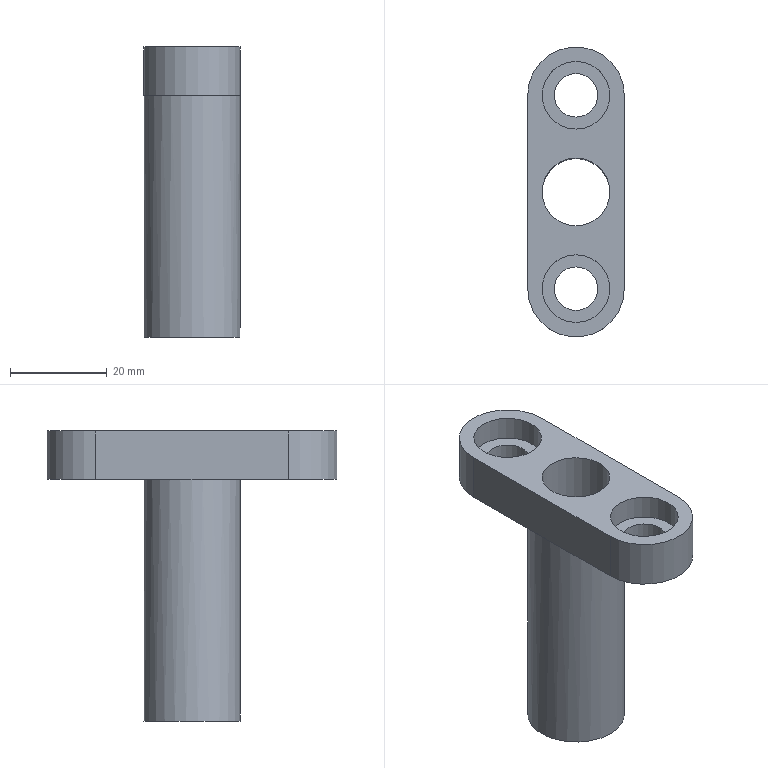Component | NX | GUIDE_BUSH | 1 solid | 16 faces | box 20 x 60 x 60 mm | volume 15438 mm3 | cylinder 8 | plane 8 | commonest cylinder face diameters 20 x3 14 x3 9 x2
STEP:
#1=CARTESIAN_POINT('',(0.,0.,0.));
#2=DIRECTION('',(0.,0.,1.));
#3=DIRECTION('',(1.,0.,0.));
#4=AXIS2_PLACEMENT_3D('',#1,#2,#3);
#5=CARTESIAN_POINT('',(40.594,327.962,290.466));
#6=VERTEX_POINT('',#5);
#7=CARTESIAN_POINT('',(40.594,332.462,290.466));
#8=DIRECTION('',(0.,0.,1.));
#9=DIRECTION('',(0.,-1.,0.));
#10=AXIS2_PLACEMENT_3D('',#7,#8,#9);
#11=CIRCLE('',#10,4.5);
#12=CARTESIAN_POINT('',(40.594,332.462,300.466));
#13=DIRECTION('',(0.,0.,-1.));
#14=DIRECTION('',(0.,1.,0.));
#15=AXIS2_PLACEMENT_3D('',#12,#13,#14);
#16=CYLINDRICAL_SURFACE('',#15,4.5);
#17=CARTESIAN_POINT('',(9.425,10.));
#18=DIRECTION('',(-1.,0.));
#19=VECTOR('',#18,1.);
#20=LINE('',#17,#19);
#21=(GEOMETRIC_REPRESENTATION_CONTEXT(2)PARAMETRIC_REPRESENTATION_CONTEXT()REPRESENTATION_CONTEXT('',''));
#22=DEFINITIONAL_REPRESENTATION('',(#20),#21);
#23=PCURVE('',#16,#22);
#24=CARTESIAN_POINT('',(40.594,332.462,290.466));
#25=DIRECTION('',(0.,0.,1.));
#26=DIRECTION('',(0.,-1.,0.));
#27=AXIS2_PLACEMENT_3D('',#24,#25,#26);
#28=PLANE('',#27);
#29=CARTESIAN_POINT('',(0.,0.));
#30=DIRECTION('',(1.,0.));
#31=AXIS2_PLACEMENT_2D('',#29,#30);
#32=CIRCLE('',#31,4.5);
#33=(GEOMETRIC_REPRESENTATION_CONTEXT(2)PARAMETRIC_REPRESENTATION_CONTEXT()REPRESENTATION_CONTEXT('',''));
#34=DEFINITIONAL_REPRESENTATION('',(#32),#33);
#35=PCURVE('',#28,#34);
#36=SURFACE_CURVE('',#11,(#23,#35),.PCURVE_S1.);
#37=EDGE_CURVE('',#6,#6,#36,.T.);
#38=ORIENTED_EDGE('',*,*,#37,.T.);
#39=CARTESIAN_POINT('',(40.594,327.962,295.466));
#40=VERTEX_POINT('',#39);
#41=CARTESIAN_POINT('',(40.594,327.962,295.466));
#42=CARTESIAN_POINT('',(40.594,327.962,290.466));
#43=B_SPLINE_CURVE_WITH_KNOTS('',1,(#41,#42),.UNSPECIFIED.,.F.,.F.,(2,2),(5.,10.),.PIECEWISE_BEZIER_KNOTS.);
#44=CARTESIAN_POINT('',(3.142,0.));
#45=DIRECTION('',(0.,1.));
#46=VECTOR('',#45,1.);
#47=LINE('',#44,#46);
#48=(GEOMETRIC_REPRESENTATION_CONTEXT(2)PARAMETRIC_REPRESENTATION_CONTEXT()REPRESENTATION_CONTEXT('',''));
#49=DEFINITIONAL_REPRESENTATION('',(#47),#48);
#50=PCURVE('',#16,#49);
#51=CARTESIAN_POINT('',(9.425,0.));
#52=DIRECTION('',(0.,1.));
#53=VECTOR('',#52,1.);
#54=LINE('',#51,#53);
#55=(GEOMETRIC_REPRESENTATION_CONTEXT(2)PARAMETRIC_REPRESENTATION_CONTEXT()REPRESENTATION_CONTEXT('',''));
#56=DEFINITIONAL_REPRESENTATION('',(#54),#55);
#57=PCURVE('',#16,#56);
#58=SEAM_CURVE('',#43,(#50,#57),.PCURVE_S1.);
#59=EDGE_CURVE('',#40,#6,#58,.T.);
#60=ORIENTED_EDGE('',*,*,#59,.F.);
#61=CARTESIAN_POINT('',(40.594,332.462,295.466));
#62=DIRECTION('',(0.,0.,1.));
#63=DIRECTION('',(0.,-1.,0.));
#64=AXIS2_PLACEMENT_3D('',#61,#62,#63);
#65=CIRCLE('',#64,4.5);
#66=CARTESIAN_POINT('',(9.425,5.));
#67=DIRECTION('',(-1.,0.));
#68=VECTOR('',#67,1.);
#69=LINE('',#66,#68);
#70=(GEOMETRIC_REPRESENTATION_CONTEXT(2)PARAMETRIC_REPRESENTATION_CONTEXT()REPRESENTATION_CONTEXT('',''));
#71=DEFINITIONAL_REPRESENTATION('',(#69),#70);
#72=PCURVE('',#16,#71);
#73=CARTESIAN_POINT('',(40.594,332.462,295.466));
#74=DIRECTION('',(0.,0.,1.));
#75=DIRECTION('',(0.,-1.,0.));
#76=AXIS2_PLACEMENT_3D('',#73,#74,#75);
#77=PLANE('',#76);
#78=CARTESIAN_POINT('',(0.,0.));
#79=DIRECTION('',(1.,0.));
#80=AXIS2_PLACEMENT_2D('',#78,#79);
#81=CIRCLE('',#80,4.5);
#82=(GEOMETRIC_REPRESENTATION_CONTEXT(2)PARAMETRIC_REPRESENTATION_CONTEXT()REPRESENTATION_CONTEXT('',''));
#83=DEFINITIONAL_REPRESENTATION('',(#81),#82);
#84=PCURVE('',#77,#83);
#85=SURFACE_CURVE('',#65,(#72,#84),.PCURVE_S1.);
#86=EDGE_CURVE('',#40,#40,#85,.T.);
#87=ORIENTED_EDGE('',*,*,#86,.F.);
#88=ORIENTED_EDGE('',*,*,#59,.T.);
#89=EDGE_LOOP('',(#38,#60,#87,#88));
#90=FACE_BOUND('',#89,.F.);
#91=ADVANCED_FACE('',(#90),#16,.F.);
#92=CARTESIAN_POINT('',(40.594,287.962,290.466));
#93=VERTEX_POINT('',#92);
#94=CARTESIAN_POINT('',(40.594,292.462,290.466));
#95=DIRECTION('',(0.,0.,1.));
#96=DIRECTION('',(0.,-1.,0.));
#97=AXIS2_PLACEMENT_3D('',#94,#95,#96);
#98=CIRCLE('',#97,4.5);
#99=CARTESIAN_POINT('',(40.594,292.462,300.466));
#100=DIRECTION('',(0.,0.,-1.));
#101=DIRECTION('',(0.,1.,0.));
#102=AXIS2_PLACEMENT_3D('',#99,#100,#101);
#103=CYLINDRICAL_SURFACE('',#102,4.5);
#104=CARTESIAN_POINT('',(9.425,10.));
#105=DIRECTION('',(-1.,0.));
#106=VECTOR('',#105,1.);
#107=LINE('',#104,#106);
#108=(GEOMETRIC_REPRESENTATION_CONTEXT(2)PARAMETRIC_REPRESENTATION_CONTEXT()REPRESENTATION_CONTEXT('',''));
#109=DEFINITIONAL_REPRESENTATION('',(#107),#108);
#110=PCURVE('',#103,#109);
#111=CARTESIAN_POINT('',(40.594,332.462,290.466));
#112=DIRECTION('',(0.,0.,1.));
#113=DIRECTION('',(0.,-1.,0.));
#114=AXIS2_PLACEMENT_3D('',#111,#112,#113);
#115=PLANE('',#114);
#116=CARTESIAN_POINT('',(40.,0.));
#117=DIRECTION('',(1.,0.));
#118=AXIS2_PLACEMENT_2D('',#116,#117);
#119=CIRCLE('',#118,4.5);
#120=(GEOMETRIC_REPRESENTATION_CONTEXT(2)PARAMETRIC_REPRESENTATION_CONTEXT()REPRESENTATION_CONTEXT('',''));
#121=DEFINITIONAL_REPRESENTATION('',(#119),#120);
#122=PCURVE('',#115,#121);
#123=SURFACE_CURVE('',#98,(#110,#122),.PCURVE_S1.);
#124=EDGE_CURVE('',#93,#93,#123,.T.);
#125=ORIENTED_EDGE('',*,*,#124,.T.);
#126=CARTESIAN_POINT('',(40.594,287.962,295.466));
#127=VERTEX_POINT('',#126);
#128=CARTESIAN_POINT('',(40.594,287.962,295.466));
#129=CARTESIAN_POINT('',(40.594,287.962,290.466));
#130=B_SPLINE_CURVE_WITH_KNOTS('',1,(#128,#129),.UNSPECIFIED.,.F.,.F.,(2,2),(5.,10.),.PIECEWISE_BEZIER_KNOTS.);
#131=CARTESIAN_POINT('',(3.142,0.));
#132=DIRECTION('',(0.,1.));
#133=VECTOR('',#132,1.);
#134=LINE('',#131,#133);
#135=(GEOMETRIC_REPRESENTATION_CONTEXT(2)PARAMETRIC_REPRESENTATION_CONTEXT()REPRESENTATION_CONTEXT('',''));
#136=DEFINITIONAL_REPRESENTATION('',(#134),#135);
#137=PCURVE('',#103,#136);
#138=CARTESIAN_POINT('',(9.425,0.));
#139=DIRECTION('',(0.,1.));
#140=VECTOR('',#139,1.);
#141=LINE('',#138,#140);
#142=(GEOMETRIC_REPRESENTATION_CONTEXT(2)PARAMETRIC_REPRESENTATION_CONTEXT()REPRESENTATION_CONTEXT('',''));
#143=DEFINITIONAL_REPRESENTATION('',(#141),#142);
#144=PCURVE('',#103,#143);
#145=SEAM_CURVE('',#130,(#137,#144),.PCURVE_S1.);
#146=EDGE_CURVE('',#127,#93,#145,.T.);
#147=ORIENTED_EDGE('',*,*,#146,.F.);
#148=CARTESIAN_POINT('',(40.594,292.462,295.466));
#149=DIRECTION('',(0.,0.,1.));
#150=DIRECTION('',(0.,-1.,0.));
#151=AXIS2_PLACEMENT_3D('',#148,#149,#150);
#152=CIRCLE('',#151,4.5);
#153=CARTESIAN_POINT('',(9.425,5.));
#154=DIRECTION('',(-1.,0.));
#155=VECTOR('',#154,1.);
#156=LINE('',#153,#155);
#157=(GEOMETRIC_REPRESENTATION_CONTEXT(2)PARAMETRIC_REPRESENTATION_CONTEXT()REPRESENTATION_CONTEXT('',''));
#158=DEFINITIONAL_REPRESENTATION('',(#156),#157);
#159=PCURVE('',#103,#158);
#160=CARTESIAN_POINT('',(40.594,292.462,295.466));
#161=DIRECTION('',(0.,0.,1.));
#162=DIRECTION('',(0.,-1.,0.));
#163=AXIS2_PLACEMENT_3D('',#160,#161,#162);
#164=PLANE('',#163);
#165=CARTESIAN_POINT('',(0.,0.));
#166=DIRECTION('',(1.,0.));
#167=AXIS2_PLACEMENT_2D('',#165,#166);
#168=CIRCLE('',#167,4.5);
#169=(GEOMETRIC_REPRESENTATION_CONTEXT(2)PARAMETRIC_REPRESENTATION_CONTEXT()REPRESENTATION_CONTEXT('',''));
#170=DEFINITIONAL_REPRESENTATION('',(#168),#169);
#171=PCURVE('',#164,#170);
#172=SURFACE_CURVE('',#152,(#159,#171),.PCURVE_S1.);
#173=EDGE_CURVE('',#127,#127,#172,.T.);
#174=ORIENTED_EDGE('',*,*,#173,.F.);
#175=ORIENTED_EDGE('',*,*,#146,.T.);
#176=EDGE_LOOP('',(#125,#147,#174,#175));
#177=FACE_BOUND('',#176,.F.);
#178=ADVANCED_FACE('',(#177),#103,.F.);
#179=CARTESIAN_POINT('',(30.594,312.462,290.466));
#180=VERTEX_POINT('',#179);
#181=CARTESIAN_POINT('',(50.594,312.462,290.466));
#182=VERTEX_POINT('',#181);
#183=CARTESIAN_POINT('',(40.594,312.462,290.466));
#184=DIRECTION('',(0.,0.,-1.));
#185=DIRECTION('',(0.,-1.,0.));
#186=AXIS2_PLACEMENT_3D('',#183,#184,#185);
#187=CIRCLE('',#186,10.);
#188=CARTESIAN_POINT('',(30.,0.));
#189=CARTESIAN_POINT('',(30.,-17.321));
#190=CARTESIAN_POINT('',(15.,-8.66));
#191=CARTESIAN_POINT('',(0.,-0.));
#192=CARTESIAN_POINT('',(15.,8.66));
#193=CARTESIAN_POINT('',(30.,17.321));
#194=CARTESIAN_POINT('',(30.,0.));
#195=(BOUNDED_CURVE()B_SPLINE_CURVE(2,(#188,#189,#190,#191,#192,#193,#194),.UNSPECIFIED.,.T.,.F.)B_SPLINE_CURVE_WITH_KNOTS((1,2,2,2,2,1),(-2.094,0.,2.094,4.189,6.283,8.378),.UNSPECIFIED.)CURVE()GEOMETRIC_REPRESENTATION_ITEM()RATIONAL_B_SPLINE_CURVE((1.,0.5,1.,0.5,1.,0.5,1.))REPRESENTATION_ITEM(''));
#196=(GEOMETRIC_REPRESENTATION_CONTEXT(2)PARAMETRIC_REPRESENTATION_CONTEXT()REPRESENTATION_CONTEXT('',''));
#197=DEFINITIONAL_REPRESENTATION('',(#195),#196);
#198=PCURVE('',#28,#197);
#199=CARTESIAN_POINT('',(40.594,312.462,240.466));
#200=DIRECTION('',(0.,0.,1.));
#201=DIRECTION('',(0.,-1.,0.));
#202=AXIS2_PLACEMENT_3D('',#199,#200,#201);
#203=CYLINDRICAL_SURFACE('',#202,10.);
#204=CARTESIAN_POINT('',(6.283,50.));
#205=DIRECTION('',(-1.,0.));
#206=VECTOR('',#205,1.);
#207=LINE('',#204,#206);
#208=(GEOMETRIC_REPRESENTATION_CONTEXT(2)PARAMETRIC_REPRESENTATION_CONTEXT()REPRESENTATION_CONTEXT('',''));
#209=DEFINITIONAL_REPRESENTATION('',(#207),#208);
#210=PCURVE('',#203,#209);
#211=SURFACE_CURVE('',#187,(#198,#210),.PCURVE_S1.);
#212=EDGE_CURVE('',#180,#182,#211,.T.);
#213=ORIENTED_EDGE('',*,*,#212,.F.);
#214=CARTESIAN_POINT('',(30.594,332.462,290.466));
#215=VERTEX_POINT('',#214);
#216=CARTESIAN_POINT('',(30.594,332.462,290.466));
#217=DIRECTION('',(0.,-1.,0.));
#218=VECTOR('',#217,1.);
#219=LINE('',#216,#218);
#220=CARTESIAN_POINT('',(0.,-10.));
#221=DIRECTION('',(1.,0.));
#222=VECTOR('',#221,1.);
#223=LINE('',#220,#222);
#224=(GEOMETRIC_REPRESENTATION_CONTEXT(2)PARAMETRIC_REPRESENTATION_CONTEXT()REPRESENTATION_CONTEXT('',''));
#225=DEFINITIONAL_REPRESENTATION('',(#223),#224);
#226=PCURVE('',#28,#225);
#227=CARTESIAN_POINT('',(30.594,332.462,300.466));
#228=DIRECTION('',(1.,0.,0.));
#229=DIRECTION('',(0.,0.,1.));
#230=AXIS2_PLACEMENT_3D('',#227,#228,#229);
#231=PLANE('',#230);
#232=CARTESIAN_POINT('',(-10.,0.));
#233=DIRECTION('',(0.,1.));
#234=VECTOR('',#233,1.);
#235=LINE('',#232,#234);
#236=(GEOMETRIC_REPRESENTATION_CONTEXT(2)PARAMETRIC_REPRESENTATION_CONTEXT()REPRESENTATION_CONTEXT('',''));
#237=DEFINITIONAL_REPRESENTATION('',(#235),#236);
#238=PCURVE('',#231,#237);
#239=SURFACE_CURVE('',#219,(#226,#238),.PCURVE_S1.);
#240=EDGE_CURVE('',#215,#180,#239,.T.);
#241=ORIENTED_EDGE('',*,*,#240,.F.);
#242=CARTESIAN_POINT('',(50.594,332.462,290.466));
#243=VERTEX_POINT('',#242);
#244=CARTESIAN_POINT('',(40.594,332.462,290.466));
#245=DIRECTION('',(0.,0.,1.));
#246=DIRECTION('',(0.,-1.,0.));
#247=AXIS2_PLACEMENT_3D('',#244,#245,#246);
#248=CIRCLE('',#247,10.);
#249=CARTESIAN_POINT('',(0.,0.));
#250=DIRECTION('',(1.,0.));
#251=AXIS2_PLACEMENT_2D('',#249,#250);
#252=CIRCLE('',#251,10.);
#253=(GEOMETRIC_REPRESENTATION_CONTEXT(2)PARAMETRIC_REPRESENTATION_CONTEXT()REPRESENTATION_CONTEXT('',''));
#254=DEFINITIONAL_REPRESENTATION('',(#252),#253);
#255=PCURVE('',#28,#254);
#256=CARTESIAN_POINT('',(40.594,332.462,300.466));
#257=DIRECTION('',(0.,0.,-1.));
#258=DIRECTION('',(0.,1.,0.));
#259=AXIS2_PLACEMENT_3D('',#256,#257,#258);
#260=CYLINDRICAL_SURFACE('',#259,10.);
#261=CARTESIAN_POINT('',(3.142,10.));
#262=DIRECTION('',(-1.,0.));
#263=VECTOR('',#262,1.);
#264=LINE('',#261,#263);
#265=(GEOMETRIC_REPRESENTATION_CONTEXT(2)PARAMETRIC_REPRESENTATION_CONTEXT()REPRESENTATION_CONTEXT('',''));
#266=DEFINITIONAL_REPRESENTATION('',(#264),#265);
#267=PCURVE('',#260,#266);
#268=SURFACE_CURVE('',#248,(#255,#267),.PCURVE_S1.);
#269=EDGE_CURVE('',#243,#215,#268,.T.);
#270=ORIENTED_EDGE('',*,*,#269,.F.);
#271=CARTESIAN_POINT('',(50.594,292.462,290.466));
#272=DIRECTION('',(-0.,1.,0.));
#273=VECTOR('',#272,1.);
#274=LINE('',#271,#273);
#275=CARTESIAN_POINT('',(40.,10.));
#276=DIRECTION('',(-1.,-0.));
#277=VECTOR('',#276,1.);
#278=LINE('',#275,#277);
#279=(GEOMETRIC_REPRESENTATION_CONTEXT(2)PARAMETRIC_REPRESENTATION_CONTEXT()REPRESENTATION_CONTEXT('',''));
#280=DEFINITIONAL_REPRESENTATION('',(#278),#279);
#281=PCURVE('',#28,#280);
#282=CARTESIAN_POINT('',(50.594,292.462,300.466));
#283=DIRECTION('',(-1.,-0.,0.));
#284=DIRECTION('',(0.,-1.,0.));
#285=AXIS2_PLACEMENT_3D('',#282,#283,#284);
#286=PLANE('',#285);
#287=CARTESIAN_POINT('',(0.,-10.));
#288=DIRECTION('',(-1.,0.));
#289=VECTOR('',#288,1.);
#290=LINE('',#287,#289);
#291=(GEOMETRIC_REPRESENTATION_CONTEXT(2)PARAMETRIC_REPRESENTATION_CONTEXT()REPRESENTATION_CONTEXT('',''));
#292=DEFINITIONAL_REPRESENTATION('',(#290),#291);
#293=PCURVE('',#286,#292);
#294=SURFACE_CURVE('',#274,(#281,#293),.PCURVE_S1.);
#295=EDGE_CURVE('',#182,#243,#294,.T.);
#296=ORIENTED_EDGE('',*,*,#295,.F.);
#297=EDGE_LOOP('',(#213,#241,#270,#296));
#298=FACE_BOUND('',#297,.T.);
#299=ORIENTED_EDGE('',*,*,#37,.T.);
#300=EDGE_LOOP('',(#299));
#301=FACE_BOUND('',#300,.T.);
#302=ADVANCED_FACE('',(#298,#301),#28,.F.);
#303=ORIENTED_EDGE('',*,*,#269,.T.);
#304=CARTESIAN_POINT('',(30.594,332.462,300.466));
#305=VERTEX_POINT('',#304);
#306=CARTESIAN_POINT('',(30.594,332.462,300.466));
#307=DIRECTION('',(0.,0.,-1.));
#308=VECTOR('',#307,1.);
#309=LINE('',#306,#308);
#310=CARTESIAN_POINT('',(-1.571,0.));
#311=DIRECTION('',(0.,1.));
#312=VECTOR('',#311,1.);
#313=LINE('',#310,#312);
#314=(GEOMETRIC_REPRESENTATION_CONTEXT(2)PARAMETRIC_REPRESENTATION_CONTEXT()REPRESENTATION_CONTEXT('',''));
#315=DEFINITIONAL_REPRESENTATION('',(#313),#314);
#316=PCURVE('',#260,#315);
#317=CARTESIAN_POINT('',(0.,0.));
#318=DIRECTION('',(-1.,0.));
#319=VECTOR('',#318,1.);
#320=LINE('',#317,#319);
#321=(GEOMETRIC_REPRESENTATION_CONTEXT(2)PARAMETRIC_REPRESENTATION_CONTEXT()REPRESENTATION_CONTEXT('',''));
#322=DEFINITIONAL_REPRESENTATION('',(#320),#321);
#323=PCURVE('',#231,#322);
#324=SURFACE_CURVE('',#309,(#316,#323),.PCURVE_S1.);
#325=EDGE_CURVE('',#305,#215,#324,.T.);
#326=ORIENTED_EDGE('',*,*,#325,.F.);
#327=CARTESIAN_POINT('',(50.594,332.462,300.466));
#328=VERTEX_POINT('',#327);
#329=CARTESIAN_POINT('',(40.594,332.462,300.466));
#330=DIRECTION('',(0.,0.,1.));
#331=DIRECTION('',(0.,-1.,0.));
#332=AXIS2_PLACEMENT_3D('',#329,#330,#331);
#333=CIRCLE('',#332,10.);
#334=CARTESIAN_POINT('',(3.142,0.));
#335=DIRECTION('',(-1.,0.));
#336=VECTOR('',#335,1.);
#337=LINE('',#334,#336);
#338=(GEOMETRIC_REPRESENTATION_CONTEXT(2)PARAMETRIC_REPRESENTATION_CONTEXT()REPRESENTATION_CONTEXT('',''));
#339=DEFINITIONAL_REPRESENTATION('',(#337),#338);
#340=PCURVE('',#260,#339);
#341=CARTESIAN_POINT('',(40.594,332.462,300.466));
#342=DIRECTION('',(0.,0.,1.));
#343=DIRECTION('',(0.,-1.,0.));
#344=AXIS2_PLACEMENT_3D('',#341,#342,#343);
#345=PLANE('',#344);
#346=CARTESIAN_POINT('',(0.,0.));
#347=DIRECTION('',(1.,0.));
#348=AXIS2_PLACEMENT_2D('',#346,#347);
#349=CIRCLE('',#348,10.);
#350=(GEOMETRIC_REPRESENTATION_CONTEXT(2)PARAMETRIC_REPRESENTATION_CONTEXT()REPRESENTATION_CONTEXT('',''));
#351=DEFINITIONAL_REPRESENTATION('',(#349),#350);
#352=PCURVE('',#345,#351);
#353=SURFACE_CURVE('',#333,(#340,#352),.PCURVE_S1.);
#354=EDGE_CURVE('',#328,#305,#353,.T.);
#355=ORIENTED_EDGE('',*,*,#354,.F.);
#356=CARTESIAN_POINT('',(50.594,332.462,300.466));
#357=DIRECTION('',(0.,0.,-1.));
#358=VECTOR('',#357,1.);
#359=LINE('',#356,#358);
#360=CARTESIAN_POINT('',(1.571,0.));
#361=DIRECTION('',(0.,1.));
#362=VECTOR('',#361,1.);
#363=LINE('',#360,#362);
#364=(GEOMETRIC_REPRESENTATION_CONTEXT(2)PARAMETRIC_REPRESENTATION_CONTEXT()REPRESENTATION_CONTEXT('',''));
#365=DEFINITIONAL_REPRESENTATION('',(#363),#364);
#366=PCURVE('',#260,#365);
#367=CARTESIAN_POINT('',(-40.,0.));
#368=DIRECTION('',(0.,-1.));
#369=VECTOR('',#368,1.);
#370=LINE('',#367,#369);
#371=(GEOMETRIC_REPRESENTATION_CONTEXT(2)PARAMETRIC_REPRESENTATION_CONTEXT()REPRESENTATION_CONTEXT('',''));
#372=DEFINITIONAL_REPRESENTATION('',(#370),#371);
#373=PCURVE('',#286,#372);
#374=SURFACE_CURVE('',#359,(#366,#373),.PCURVE_S1.);
#375=EDGE_CURVE('',#328,#243,#374,.T.);
#376=ORIENTED_EDGE('',*,*,#375,.T.);
#377=EDGE_LOOP('',(#303,#326,#355,#376));
#378=FACE_BOUND('',#377,.T.);
#379=ADVANCED_FACE('',(#378),#260,.T.);
#380=ORIENTED_EDGE('',*,*,#240,.T.);
#381=CARTESIAN_POINT('',(30.594,292.462,290.466));
#382=VERTEX_POINT('',#381);
#383=CARTESIAN_POINT('',(30.594,332.462,290.466));
#384=DIRECTION('',(0.,-1.,0.));
#385=VECTOR('',#384,1.);
#386=LINE('',#383,#385);
#387=CARTESIAN_POINT('',(-10.,0.));
#388=DIRECTION('',(0.,1.));
#389=VECTOR('',#388,1.);
#390=LINE('',#387,#389);
#391=(GEOMETRIC_REPRESENTATION_CONTEXT(2)PARAMETRIC_REPRESENTATION_CONTEXT()REPRESENTATION_CONTEXT('',''));
#392=DEFINITIONAL_REPRESENTATION('',(#390),#391);
#393=PCURVE('',#231,#392);
#394=CARTESIAN_POINT('',(0.,-10.));
#395=DIRECTION('',(1.,0.));
#396=VECTOR('',#395,1.);
#397=LINE('',#394,#396);
#398=(GEOMETRIC_REPRESENTATION_CONTEXT(2)PARAMETRIC_REPRESENTATION_CONTEXT()REPRESENTATION_CONTEXT('',''));
#399=DEFINITIONAL_REPRESENTATION('',(#397),#398);
#400=PCURVE('',#115,#399);
#401=SURFACE_CURVE('',#386,(#393,#400),.PCURVE_S1.);
#402=EDGE_CURVE('',#180,#382,#401,.T.);
#403=ORIENTED_EDGE('',*,*,#402,.T.);
#404=CARTESIAN_POINT('',(30.594,292.462,300.466));
#405=VERTEX_POINT('',#404);
#406=CARTESIAN_POINT('',(30.594,292.462,300.466));
#407=DIRECTION('',(0.,0.,-1.));
#408=VECTOR('',#407,1.);
#409=LINE('',#406,#408);
#410=CARTESIAN_POINT('',(0.,40.));
#411=DIRECTION('',(-1.,0.));
#412=VECTOR('',#411,1.);
#413=LINE('',#410,#412);
#414=(GEOMETRIC_REPRESENTATION_CONTEXT(2)PARAMETRIC_REPRESENTATION_CONTEXT()REPRESENTATION_CONTEXT('',''));
#415=DEFINITIONAL_REPRESENTATION('',(#413),#414);
#416=PCURVE('',#231,#415);
#417=CARTESIAN_POINT('',(40.594,292.462,300.466));
#418=DIRECTION('',(0.,0.,-1.));
#419=DIRECTION('',(0.,1.,0.));
#420=AXIS2_PLACEMENT_3D('',#417,#418,#419);
#421=CYLINDRICAL_SURFACE('',#420,10.);
#422=CARTESIAN_POINT('',(4.712,0.));
#423=DIRECTION('',(0.,1.));
#424=VECTOR('',#423,1.);
#425=LINE('',#422,#424);
#426=(GEOMETRIC_REPRESENTATION_CONTEXT(2)PARAMETRIC_REPRESENTATION_CONTEXT()REPRESENTATION_CONTEXT('',''));
#427=DEFINITIONAL_REPRESENTATION('',(#425),#426);
#428=PCURVE('',#421,#427);
#429=SURFACE_CURVE('',#409,(#416,#428),.PCURVE_S1.);
#430=EDGE_CURVE('',#405,#382,#429,.T.);
#431=ORIENTED_EDGE('',*,*,#430,.F.);
#432=CARTESIAN_POINT('',(30.594,332.462,300.466));
#433=DIRECTION('',(0.,-1.,0.));
#434=VECTOR('',#433,1.);
#435=LINE('',#432,#434);
#436=CARTESIAN_POINT('',(0.,0.));
#437=DIRECTION('',(0.,1.));
#438=VECTOR('',#437,1.);
#439=LINE('',#436,#438);
#440=(GEOMETRIC_REPRESENTATION_CONTEXT(2)PARAMETRIC_REPRESENTATION_CONTEXT()REPRESENTATION_CONTEXT('',''));
#441=DEFINITIONAL_REPRESENTATION('',(#439),#440);
#442=PCURVE('',#231,#441);
#443=CARTESIAN_POINT('',(0.,-10.));
#444=DIRECTION('',(1.,0.));
#445=VECTOR('',#444,1.);
#446=LINE('',#443,#445);
#447=(GEOMETRIC_REPRESENTATION_CONTEXT(2)PARAMETRIC_REPRESENTATION_CONTEXT()REPRESENTATION_CONTEXT('',''));
#448=DEFINITIONAL_REPRESENTATION('',(#446),#447);
#449=PCURVE('',#345,#448);
#450=SURFACE_CURVE('',#435,(#442,#449),.PCURVE_S1.);
#451=EDGE_CURVE('',#305,#405,#450,.T.);
#452=ORIENTED_EDGE('',*,*,#451,.F.);
#453=ORIENTED_EDGE('',*,*,#325,.T.);
#454=EDGE_LOOP('',(#380,#403,#431,#452,#453));
#455=FACE_BOUND('',#454,.T.);
#456=ADVANCED_FACE('',(#455),#231,.F.);
#457=CARTESIAN_POINT('',(50.594,292.462,290.466));
#458=VERTEX_POINT('',#457);
#459=CARTESIAN_POINT('',(40.594,292.462,290.466));
#460=DIRECTION('',(0.,0.,1.));
#461=DIRECTION('',(0.,-1.,0.));
#462=AXIS2_PLACEMENT_3D('',#459,#460,#461);
#463=CIRCLE('',#462,10.);
#464=CARTESIAN_POINT('',(9.425,10.));
#465=DIRECTION('',(-1.,0.));
#466=VECTOR('',#465,1.);
#467=LINE('',#464,#466);
#468=(GEOMETRIC_REPRESENTATION_CONTEXT(2)PARAMETRIC_REPRESENTATION_CONTEXT()REPRESENTATION_CONTEXT('',''));
#469=DEFINITIONAL_REPRESENTATION('',(#467),#468);
#470=PCURVE('',#421,#469);
#471=CARTESIAN_POINT('',(40.,0.));
#472=DIRECTION('',(1.,0.));
#473=AXIS2_PLACEMENT_2D('',#471,#472);
#474=CIRCLE('',#473,10.);
#475=(GEOMETRIC_REPRESENTATION_CONTEXT(2)PARAMETRIC_REPRESENTATION_CONTEXT()REPRESENTATION_CONTEXT('',''));
#476=DEFINITIONAL_REPRESENTATION('',(#474),#475);
#477=PCURVE('',#115,#476);
#478=SURFACE_CURVE('',#463,(#470,#477),.PCURVE_S1.);
#479=EDGE_CURVE('',#382,#458,#478,.T.);
#480=ORIENTED_EDGE('',*,*,#479,.T.);
#481=CARTESIAN_POINT('',(50.594,292.462,300.466));
#482=VERTEX_POINT('',#481);
#483=CARTESIAN_POINT('',(50.594,292.462,300.466));
#484=DIRECTION('',(0.,0.,-1.));
#485=VECTOR('',#484,1.);
#486=LINE('',#483,#485);
#487=CARTESIAN_POINT('',(1.571,0.));
#488=DIRECTION('',(0.,1.));
#489=VECTOR('',#488,1.);
#490=LINE('',#487,#489);
#491=(GEOMETRIC_REPRESENTATION_CONTEXT(2)PARAMETRIC_REPRESENTATION_CONTEXT()REPRESENTATION_CONTEXT('',''));
#492=DEFINITIONAL_REPRESENTATION('',(#490),#491);
#493=PCURVE('',#421,#492);
#494=CARTESIAN_POINT('',(0.,0.));
#495=DIRECTION('',(0.,-1.));
#496=VECTOR('',#495,1.);
#497=LINE('',#494,#496);
#498=(GEOMETRIC_REPRESENTATION_CONTEXT(2)PARAMETRIC_REPRESENTATION_CONTEXT()REPRESENTATION_CONTEXT('',''));
#499=DEFINITIONAL_REPRESENTATION('',(#497),#498);
#500=PCURVE('',#286,#499);
#501=SURFACE_CURVE('',#486,(#493,#500),.PCURVE_S1.);
#502=EDGE_CURVE('',#482,#458,#501,.T.);
#503=ORIENTED_EDGE('',*,*,#502,.F.);
#504=CARTESIAN_POINT('',(40.594,292.462,300.466));
#505=DIRECTION('',(0.,0.,1.));
#506=DIRECTION('',(0.,-1.,0.));
#507=AXIS2_PLACEMENT_3D('',#504,#505,#506);
#508=CIRCLE('',#507,10.);
#509=CARTESIAN_POINT('',(9.425,0.));
#510=DIRECTION('',(-1.,0.));
#511=VECTOR('',#510,1.);
#512=LINE('',#509,#511);
#513=(GEOMETRIC_REPRESENTATION_CONTEXT(2)PARAMETRIC_REPRESENTATION_CONTEXT()REPRESENTATION_CONTEXT('',''));
#514=DEFINITIONAL_REPRESENTATION('',(#512),#513);
#515=PCURVE('',#421,#514);
#516=CARTESIAN_POINT('',(40.,0.));
#517=DIRECTION('',(1.,0.));
#518=AXIS2_PLACEMENT_2D('',#516,#517);
#519=CIRCLE('',#518,10.);
#520=(GEOMETRIC_REPRESENTATION_CONTEXT(2)PARAMETRIC_REPRESENTATION_CONTEXT()REPRESENTATION_CONTEXT('',''));
#521=DEFINITIONAL_REPRESENTATION('',(#519),#520);
#522=PCURVE('',#345,#521);
#523=SURFACE_CURVE('',#508,(#515,#522),.PCURVE_S1.);
#524=EDGE_CURVE('',#405,#482,#523,.T.);
#525=ORIENTED_EDGE('',*,*,#524,.F.);
#526=ORIENTED_EDGE('',*,*,#430,.T.);
#527=EDGE_LOOP('',(#480,#503,#525,#526));
#528=FACE_BOUND('',#527,.T.);
#529=ADVANCED_FACE('',(#528),#421,.T.);
#530=CARTESIAN_POINT('',(40.594,305.462,300.466));
#531=VERTEX_POINT('',#530);
#532=CARTESIAN_POINT('',(40.594,312.462,300.466));
#533=DIRECTION('',(0.,0.,1.));
#534=DIRECTION('',(0.,-1.,0.));
#535=AXIS2_PLACEMENT_3D('',#532,#533,#534);
#536=CIRCLE('',#535,7.);
#537=CARTESIAN_POINT('',(40.594,312.462,300.466));
#538=DIRECTION('',(0.,0.,-1.));
#539=DIRECTION('',(0.,1.,0.));
#540=AXIS2_PLACEMENT_3D('',#537,#538,#539);
#541=CYLINDRICAL_SURFACE('',#540,7.);
#542=CARTESIAN_POINT('',(9.425,0.));
#543=DIRECTION('',(-1.,0.));
#544=VECTOR('',#543,1.);
#545=LINE('',#542,#544);
#546=(GEOMETRIC_REPRESENTATION_CONTEXT(2)PARAMETRIC_REPRESENTATION_CONTEXT()REPRESENTATION_CONTEXT('',''));
#547=DEFINITIONAL_REPRESENTATION('',(#545),#546);
#548=PCURVE('',#541,#547);
#549=CARTESIAN_POINT('',(20.,0.));
#550=DIRECTION('',(1.,0.));
#551=AXIS2_PLACEMENT_2D('',#549,#550);
#552=CIRCLE('',#551,7.);
#553=(GEOMETRIC_REPRESENTATION_CONTEXT(2)PARAMETRIC_REPRESENTATION_CONTEXT()REPRESENTATION_CONTEXT('',''));
#554=DEFINITIONAL_REPRESENTATION('',(#552),#553);
#555=PCURVE('',#345,#554);
#556=SURFACE_CURVE('',#536,(#548,#555),.PCURVE_S1.);
#557=EDGE_CURVE('',#531,#531,#556,.T.);
#558=ORIENTED_EDGE('',*,*,#557,.F.);
#559=CARTESIAN_POINT('',(40.594,305.462,240.466));
#560=VERTEX_POINT('',#559);
#561=CARTESIAN_POINT('',(40.594,305.462,300.466));
#562=CARTESIAN_POINT('',(40.594,305.462,240.466));
#563=B_SPLINE_CURVE_WITH_KNOTS('',1,(#561,#562),.UNSPECIFIED.,.F.,.F.,(2,2),(0.,60.),.PIECEWISE_BEZIER_KNOTS.);
#564=CARTESIAN_POINT('',(9.425,0.));
#565=DIRECTION('',(0.,1.));
#566=VECTOR('',#565,1.);
#567=LINE('',#564,#566);
#568=(GEOMETRIC_REPRESENTATION_CONTEXT(2)PARAMETRIC_REPRESENTATION_CONTEXT()REPRESENTATION_CONTEXT('',''));
#569=DEFINITIONAL_REPRESENTATION('',(#567),#568);
#570=PCURVE('',#541,#569);
#571=CARTESIAN_POINT('',(3.142,0.));
#572=DIRECTION('',(0.,1.));
#573=VECTOR('',#572,1.);
#574=LINE('',#571,#573);
#575=(GEOMETRIC_REPRESENTATION_CONTEXT(2)PARAMETRIC_REPRESENTATION_CONTEXT()REPRESENTATION_CONTEXT('',''));
#576=DEFINITIONAL_REPRESENTATION('',(#574),#575);
#577=PCURVE('',#541,#576);
#578=SEAM_CURVE('',#563,(#570,#577),.PCURVE_S1.);
#579=EDGE_CURVE('',#531,#560,#578,.T.);
#580=ORIENTED_EDGE('',*,*,#579,.T.);
#581=CARTESIAN_POINT('',(40.594,312.462,240.466));
#582=DIRECTION('',(0.,0.,-1.));
#583=DIRECTION('',(0.,-1.,0.));
#584=AXIS2_PLACEMENT_3D('',#581,#582,#583);
#585=CIRCLE('',#584,7.);
#586=CARTESIAN_POINT('',(3.142,60.));
#587=DIRECTION('',(1.,0.));
#588=VECTOR('',#587,1.);
#589=LINE('',#586,#588);
#590=(GEOMETRIC_REPRESENTATION_CONTEXT(2)PARAMETRIC_REPRESENTATION_CONTEXT()REPRESENTATION_CONTEXT('',''));
#591=DEFINITIONAL_REPRESENTATION('',(#589),#590);
#592=PCURVE('',#541,#591);
#593=CARTESIAN_POINT('',(40.594,312.462,240.466));
#594=DIRECTION('',(0.,0.,-1.));
#595=DIRECTION('',(0.,1.,0.));
#596=AXIS2_PLACEMENT_3D('',#593,#594,#595);
#597=PLANE('',#596);
#598=CARTESIAN_POINT('',(0.,0.));
#599=DIRECTION('',(-1.,0.));
#600=AXIS2_PLACEMENT_2D('',#598,#599);
#601=CIRCLE('',#600,7.);
#602=(GEOMETRIC_REPRESENTATION_CONTEXT(2)PARAMETRIC_REPRESENTATION_CONTEXT()REPRESENTATION_CONTEXT('',''));
#603=DEFINITIONAL_REPRESENTATION('',(#601),#602);
#604=PCURVE('',#597,#603);
#605=SURFACE_CURVE('',#585,(#592,#604),.PCURVE_S1.);
#606=EDGE_CURVE('',#560,#560,#605,.T.);
#607=ORIENTED_EDGE('',*,*,#606,.F.);
#608=ORIENTED_EDGE('',*,*,#579,.F.);
#609=EDGE_LOOP('',(#558,#580,#607,#608));
#610=FACE_BOUND('',#609,.F.);
#611=ADVANCED_FACE('',(#610),#541,.F.);
#612=CARTESIAN_POINT('',(50.594,292.462,290.466));
#613=DIRECTION('',(-0.,1.,0.));
#614=VECTOR('',#613,1.);
#615=LINE('',#612,#614);
#616=CARTESIAN_POINT('',(0.,-10.));
#617=DIRECTION('',(-1.,0.));
#618=VECTOR('',#617,1.);
#619=LINE('',#616,#618);
#620=(GEOMETRIC_REPRESENTATION_CONTEXT(2)PARAMETRIC_REPRESENTATION_CONTEXT()REPRESENTATION_CONTEXT('',''));
#621=DEFINITIONAL_REPRESENTATION('',(#619),#620);
#622=PCURVE('',#286,#621);
#623=CARTESIAN_POINT('',(40.,10.));
#624=DIRECTION('',(-1.,-0.));
#625=VECTOR('',#624,1.);
#626=LINE('',#623,#625);
#627=(GEOMETRIC_REPRESENTATION_CONTEXT(2)PARAMETRIC_REPRESENTATION_CONTEXT()REPRESENTATION_CONTEXT('',''));
#628=DEFINITIONAL_REPRESENTATION('',(#626),#627);
#629=PCURVE('',#115,#628);
#630=SURFACE_CURVE('',#615,(#622,#629),.PCURVE_S1.);
#631=EDGE_CURVE('',#458,#182,#630,.T.);
#632=ORIENTED_EDGE('',*,*,#631,.T.);
#633=ORIENTED_EDGE('',*,*,#295,.T.);
#634=ORIENTED_EDGE('',*,*,#375,.F.);
#635=CARTESIAN_POINT('',(50.594,292.462,300.466));
#636=DIRECTION('',(-0.,1.,0.));
#637=VECTOR('',#636,1.);
#638=LINE('',#635,#637);
#639=CARTESIAN_POINT('',(0.,0.));
#640=DIRECTION('',(-1.,0.));
#641=VECTOR('',#640,1.);
#642=LINE('',#639,#641);
#643=(GEOMETRIC_REPRESENTATION_CONTEXT(2)PARAMETRIC_REPRESENTATION_CONTEXT()REPRESENTATION_CONTEXT('',''));
#644=DEFINITIONAL_REPRESENTATION('',(#642),#643);
#645=PCURVE('',#286,#644);
#646=CARTESIAN_POINT('',(40.,10.));
#647=DIRECTION('',(-1.,-0.));
#648=VECTOR('',#647,1.);
#649=LINE('',#646,#648);
#650=(GEOMETRIC_REPRESENTATION_CONTEXT(2)PARAMETRIC_REPRESENTATION_CONTEXT()REPRESENTATION_CONTEXT('',''));
#651=DEFINITIONAL_REPRESENTATION('',(#649),#650);
#652=PCURVE('',#345,#651);
#653=SURFACE_CURVE('',#638,(#645,#652),.PCURVE_S1.);
#654=EDGE_CURVE('',#482,#328,#653,.T.);
#655=ORIENTED_EDGE('',*,*,#654,.F.);
#656=ORIENTED_EDGE('',*,*,#502,.T.);
#657=EDGE_LOOP('',(#632,#633,#634,#655,#656));
#658=FACE_BOUND('',#657,.T.);
#659=ADVANCED_FACE('',(#658),#286,.F.);
#660=CARTESIAN_POINT('',(40.594,325.462,300.466));
#661=VERTEX_POINT('',#660);
#662=CARTESIAN_POINT('',(40.594,332.462,300.466));
#663=DIRECTION('',(0.,0.,1.));
#664=DIRECTION('',(0.,-1.,0.));
#665=AXIS2_PLACEMENT_3D('',#662,#663,#664);
#666=CIRCLE('',#665,7.);
#667=CARTESIAN_POINT('',(0.,0.));
#668=DIRECTION('',(1.,0.));
#669=AXIS2_PLACEMENT_2D('',#667,#668);
#670=CIRCLE('',#669,7.);
#671=(GEOMETRIC_REPRESENTATION_CONTEXT(2)PARAMETRIC_REPRESENTATION_CONTEXT()REPRESENTATION_CONTEXT('',''));
#672=DEFINITIONAL_REPRESENTATION('',(#670),#671);
#673=PCURVE('',#345,#672);
#674=CARTESIAN_POINT('',(40.594,332.462,295.466));
#675=DIRECTION('',(0.,0.,1.));
#676=DIRECTION('',(0.,-1.,0.));
#677=AXIS2_PLACEMENT_3D('',#674,#675,#676);
#678=CYLINDRICAL_SURFACE('',#677,7.);
#679=CARTESIAN_POINT('',(0.,5.));
#680=DIRECTION('',(1.,0.));
#681=VECTOR('',#680,1.);
#682=LINE('',#679,#681);
#683=(GEOMETRIC_REPRESENTATION_CONTEXT(2)PARAMETRIC_REPRESENTATION_CONTEXT()REPRESENTATION_CONTEXT('',''));
#684=DEFINITIONAL_REPRESENTATION('',(#682),#683);
#685=PCURVE('',#678,#684);
#686=SURFACE_CURVE('',#666,(#673,#685),.PCURVE_S1.);
#687=EDGE_CURVE('',#661,#661,#686,.T.);
#688=ORIENTED_EDGE('',*,*,#687,.F.);
#689=EDGE_LOOP('',(#688));
#690=FACE_BOUND('',#689,.T.);
#691=CARTESIAN_POINT('',(40.594,285.462,300.466));
#692=VERTEX_POINT('',#691);
#693=CARTESIAN_POINT('',(40.594,292.462,300.466));
#694=DIRECTION('',(0.,0.,1.));
#695=DIRECTION('',(0.,-1.,0.));
#696=AXIS2_PLACEMENT_3D('',#693,#694,#695);
#697=CIRCLE('',#696,7.);
#698=CARTESIAN_POINT('',(40.,0.));
#699=DIRECTION('',(1.,0.));
#700=AXIS2_PLACEMENT_2D('',#698,#699);
#701=CIRCLE('',#700,7.);
#702=(GEOMETRIC_REPRESENTATION_CONTEXT(2)PARAMETRIC_REPRESENTATION_CONTEXT()REPRESENTATION_CONTEXT('',''));
#703=DEFINITIONAL_REPRESENTATION('',(#701),#702);
#704=PCURVE('',#345,#703);
#705=CARTESIAN_POINT('',(40.594,292.462,295.466));
#706=DIRECTION('',(0.,0.,1.));
#707=DIRECTION('',(0.,-1.,0.));
#708=AXIS2_PLACEMENT_3D('',#705,#706,#707);
#709=CYLINDRICAL_SURFACE('',#708,7.);
#710=CARTESIAN_POINT('',(0.,5.));
#711=DIRECTION('',(1.,0.));
#712=VECTOR('',#711,1.);
#713=LINE('',#710,#712);
#714=(GEOMETRIC_REPRESENTATION_CONTEXT(2)PARAMETRIC_REPRESENTATION_CONTEXT()REPRESENTATION_CONTEXT('',''));
#715=DEFINITIONAL_REPRESENTATION('',(#713),#714);
#716=PCURVE('',#709,#715);
#717=SURFACE_CURVE('',#697,(#704,#716),.PCURVE_S1.);
#718=EDGE_CURVE('',#692,#692,#717,.T.);
#719=ORIENTED_EDGE('',*,*,#718,.F.);
#720=EDGE_LOOP('',(#719));
#721=FACE_BOUND('',#720,.T.);
#722=ORIENTED_EDGE('',*,*,#354,.T.);
#723=ORIENTED_EDGE('',*,*,#451,.T.);
#724=ORIENTED_EDGE('',*,*,#524,.T.);
#725=ORIENTED_EDGE('',*,*,#654,.T.);
#726=EDGE_LOOP('',(#722,#723,#724,#725));
#727=FACE_BOUND('',#726,.T.);
#728=ORIENTED_EDGE('',*,*,#557,.F.);
#729=EDGE_LOOP('',(#728));
#730=FACE_BOUND('',#729,.T.);
#731=ADVANCED_FACE('',(#690,#721,#727,#730),#345,.T.);
#732=CARTESIAN_POINT('',(40.594,302.462,290.466));
#733=VERTEX_POINT('',#732);
#734=CARTESIAN_POINT('',(40.594,312.462,290.466));
#735=DIRECTION('',(0.,0.,-1.));
#736=DIRECTION('',(0.,-1.,0.));
#737=AXIS2_PLACEMENT_3D('',#734,#735,#736);
#738=CIRCLE('',#737,10.);
#739=CARTESIAN_POINT('',(30.,0.));
#740=CARTESIAN_POINT('',(30.,-17.321));
#741=CARTESIAN_POINT('',(15.,-8.66));
#742=CARTESIAN_POINT('',(0.,-0.));
#743=CARTESIAN_POINT('',(15.,8.66));
#744=CARTESIAN_POINT('',(30.,17.321));
#745=CARTESIAN_POINT('',(30.,0.));
#746=(BOUNDED_CURVE()B_SPLINE_CURVE(2,(#739,#740,#741,#742,#743,#744,#745),.UNSPECIFIED.,.T.,.F.)B_SPLINE_CURVE_WITH_KNOTS((1,2,2,2,2,1),(-2.094,0.,2.094,4.189,6.283,8.378),.UNSPECIFIED.)CURVE()GEOMETRIC_REPRESENTATION_ITEM()RATIONAL_B_SPLINE_CURVE((1.,0.5,1.,0.5,1.,0.5,1.))REPRESENTATION_ITEM(''));
#747=(GEOMETRIC_REPRESENTATION_CONTEXT(2)PARAMETRIC_REPRESENTATION_CONTEXT()REPRESENTATION_CONTEXT('',''));
#748=DEFINITIONAL_REPRESENTATION('',(#746),#747);
#749=PCURVE('',#115,#748);
#750=CARTESIAN_POINT('',(6.283,50.));
#751=DIRECTION('',(-1.,0.));
#752=VECTOR('',#751,1.);
#753=LINE('',#750,#752);
#754=(GEOMETRIC_REPRESENTATION_CONTEXT(2)PARAMETRIC_REPRESENTATION_CONTEXT()REPRESENTATION_CONTEXT('',''));
#755=DEFINITIONAL_REPRESENTATION('',(#753),#754);
#756=PCURVE('',#203,#755);
#757=SURFACE_CURVE('',#738,(#749,#756),.PCURVE_S1.);
#758=EDGE_CURVE('',#182,#733,#757,.T.);
#759=ORIENTED_EDGE('',*,*,#758,.F.);
#760=ORIENTED_EDGE('',*,*,#631,.F.);
#761=ORIENTED_EDGE('',*,*,#479,.F.);
#762=ORIENTED_EDGE('',*,*,#402,.F.);
#763=CARTESIAN_POINT('',(40.594,312.462,290.466));
#764=DIRECTION('',(0.,0.,-1.));
#765=DIRECTION('',(0.,-1.,0.));
#766=AXIS2_PLACEMENT_3D('',#763,#764,#765);
#767=CIRCLE('',#766,10.);
#768=CARTESIAN_POINT('',(30.,0.));
#769=CARTESIAN_POINT('',(30.,-17.321));
#770=CARTESIAN_POINT('',(15.,-8.66));
#771=CARTESIAN_POINT('',(0.,-0.));
#772=CARTESIAN_POINT('',(15.,8.66));
#773=CARTESIAN_POINT('',(30.,17.321));
#774=CARTESIAN_POINT('',(30.,0.));
#775=(BOUNDED_CURVE()B_SPLINE_CURVE(2,(#768,#769,#770,#771,#772,#773,#774),.UNSPECIFIED.,.T.,.F.)B_SPLINE_CURVE_WITH_KNOTS((1,2,2,2,2,1),(-2.094,0.,2.094,4.189,6.283,8.378),.UNSPECIFIED.)CURVE()GEOMETRIC_REPRESENTATION_ITEM()RATIONAL_B_SPLINE_CURVE((1.,0.5,1.,0.5,1.,0.5,1.))REPRESENTATION_ITEM(''));
#776=(GEOMETRIC_REPRESENTATION_CONTEXT(2)PARAMETRIC_REPRESENTATION_CONTEXT()REPRESENTATION_CONTEXT('',''));
#777=DEFINITIONAL_REPRESENTATION('',(#775),#776);
#778=PCURVE('',#115,#777);
#779=CARTESIAN_POINT('',(12.566,50.));
#780=DIRECTION('',(-1.,0.));
#781=VECTOR('',#780,1.);
#782=LINE('',#779,#781);
#783=(GEOMETRIC_REPRESENTATION_CONTEXT(2)PARAMETRIC_REPRESENTATION_CONTEXT()REPRESENTATION_CONTEXT('',''));
#784=DEFINITIONAL_REPRESENTATION('',(#782),#783);
#785=PCURVE('',#203,#784);
#786=SURFACE_CURVE('',#767,(#778,#785),.PCURVE_S1.);
#787=EDGE_CURVE('',#733,#180,#786,.T.);
#788=ORIENTED_EDGE('',*,*,#787,.F.);
#789=EDGE_LOOP('',(#759,#760,#761,#762,#788));
#790=FACE_BOUND('',#789,.T.);
#791=ORIENTED_EDGE('',*,*,#124,.T.);
#792=EDGE_LOOP('',(#791));
#793=FACE_BOUND('',#792,.T.);
#794=ADVANCED_FACE('',(#790,#793),#115,.F.);
#795=CARTESIAN_POINT('',(40.594,302.462,240.466));
#796=VERTEX_POINT('',#795);
#797=CARTESIAN_POINT('',(40.594,312.462,240.466));
#798=DIRECTION('',(0.,0.,-1.));
#799=DIRECTION('',(0.,-1.,0.));
#800=AXIS2_PLACEMENT_3D('',#797,#798,#799);
#801=CIRCLE('',#800,10.);
#802=CARTESIAN_POINT('',(6.283,0.));
#803=DIRECTION('',(-1.,0.));
#804=VECTOR('',#803,1.);
#805=LINE('',#802,#804);
#806=(GEOMETRIC_REPRESENTATION_CONTEXT(2)PARAMETRIC_REPRESENTATION_CONTEXT()REPRESENTATION_CONTEXT('',''));
#807=DEFINITIONAL_REPRESENTATION('',(#805),#806);
#808=PCURVE('',#203,#807);
#809=CARTESIAN_POINT('',(0.,0.));
#810=DIRECTION('',(-1.,0.));
#811=AXIS2_PLACEMENT_2D('',#809,#810);
#812=CIRCLE('',#811,10.);
#813=(GEOMETRIC_REPRESENTATION_CONTEXT(2)PARAMETRIC_REPRESENTATION_CONTEXT()REPRESENTATION_CONTEXT('',''));
#814=DEFINITIONAL_REPRESENTATION('',(#812),#813);
#815=PCURVE('',#597,#814);
#816=SURFACE_CURVE('',#801,(#808,#815),.PCURVE_S1.);
#817=EDGE_CURVE('',#796,#796,#816,.T.);
#818=ORIENTED_EDGE('',*,*,#817,.F.);
#819=CARTESIAN_POINT('',(40.594,302.462,240.466));
#820=CARTESIAN_POINT('',(40.594,302.462,290.466));
#821=B_SPLINE_CURVE_WITH_KNOTS('',1,(#819,#820),.UNSPECIFIED.,.F.,.F.,(2,2),(0.,50.),.PIECEWISE_BEZIER_KNOTS.);
#822=CARTESIAN_POINT('',(6.283,0.));
#823=DIRECTION('',(0.,1.));
#824=VECTOR('',#823,1.);
#825=LINE('',#822,#824);
#826=(GEOMETRIC_REPRESENTATION_CONTEXT(2)PARAMETRIC_REPRESENTATION_CONTEXT()REPRESENTATION_CONTEXT('',''));
#827=DEFINITIONAL_REPRESENTATION('',(#825),#826);
#828=PCURVE('',#203,#827);
#829=CARTESIAN_POINT('',(0.,0.));
#830=DIRECTION('',(0.,1.));
#831=VECTOR('',#830,1.);
#832=LINE('',#829,#831);
#833=(GEOMETRIC_REPRESENTATION_CONTEXT(2)PARAMETRIC_REPRESENTATION_CONTEXT()REPRESENTATION_CONTEXT('',''));
#834=DEFINITIONAL_REPRESENTATION('',(#832),#833);
#835=PCURVE('',#203,#834);
#836=SEAM_CURVE('',#821,(#828,#835),.PCURVE_S1.);
#837=EDGE_CURVE('',#796,#733,#836,.T.);
#838=ORIENTED_EDGE('',*,*,#837,.T.);
#839=ORIENTED_EDGE('',*,*,#787,.T.);
#840=ORIENTED_EDGE('',*,*,#212,.T.);
#841=ORIENTED_EDGE('',*,*,#758,.T.);
#842=ORIENTED_EDGE('',*,*,#837,.F.);
#843=EDGE_LOOP('',(#818,#838,#839,#840,#841,#842));
#844=FACE_BOUND('',#843,.T.);
#845=ADVANCED_FACE('',(#844),#203,.T.);
#846=ORIENTED_EDGE('',*,*,#817,.T.);
#847=EDGE_LOOP('',(#846));
#848=FACE_BOUND('',#847,.T.);
#849=ORIENTED_EDGE('',*,*,#606,.F.);
#850=EDGE_LOOP('',(#849));
#851=FACE_BOUND('',#850,.T.);
#852=ADVANCED_FACE('',(#848,#851),#597,.T.);
#853=CARTESIAN_POINT('',(40.594,285.462,295.466));
#854=VERTEX_POINT('',#853);
#855=CARTESIAN_POINT('',(40.594,292.462,295.466));
#856=DIRECTION('',(0.,0.,-1.));
#857=DIRECTION('',(0.,-1.,0.));
#858=AXIS2_PLACEMENT_3D('',#855,#856,#857);
#859=CIRCLE('',#858,7.);
#860=CARTESIAN_POINT('',(6.283,0.));
#861=DIRECTION('',(-1.,0.));
#862=VECTOR('',#861,1.);
#863=LINE('',#860,#862);
#864=(GEOMETRIC_REPRESENTATION_CONTEXT(2)PARAMETRIC_REPRESENTATION_CONTEXT()REPRESENTATION_CONTEXT('',''));
#865=DEFINITIONAL_REPRESENTATION('',(#863),#864);
#866=PCURVE('',#709,#865);
#867=CARTESIAN_POINT('',(7.,0.));
#868=CARTESIAN_POINT('',(7.,-12.124));
#869=CARTESIAN_POINT('',(-3.5,-6.062));
#870=CARTESIAN_POINT('',(-14.,-0.));
#871=CARTESIAN_POINT('',(-3.5,6.062));
#872=CARTESIAN_POINT('',(7.,12.124));
#873=CARTESIAN_POINT('',(7.,0.));
#874=(BOUNDED_CURVE()B_SPLINE_CURVE(2,(#867,#868,#869,#870,#871,#872,#873),.UNSPECIFIED.,.T.,.F.)B_SPLINE_CURVE_WITH_KNOTS((1,2,2,2,2,1),(-2.094,0.,2.094,4.189,6.283,8.378),.UNSPECIFIED.)CURVE()GEOMETRIC_REPRESENTATION_ITEM()RATIONAL_B_SPLINE_CURVE((1.,0.5,1.,0.5,1.,0.5,1.))REPRESENTATION_ITEM(''));
#875=(GEOMETRIC_REPRESENTATION_CONTEXT(2)PARAMETRIC_REPRESENTATION_CONTEXT()REPRESENTATION_CONTEXT('',''));
#876=DEFINITIONAL_REPRESENTATION('',(#874),#875);
#877=PCURVE('',#164,#876);
#878=SURFACE_CURVE('',#859,(#866,#877),.PCURVE_S1.);
#879=EDGE_CURVE('',#854,#854,#878,.T.);
#880=ORIENTED_EDGE('',*,*,#879,.F.);
#881=CARTESIAN_POINT('',(40.594,285.462,295.466));
#882=CARTESIAN_POINT('',(40.594,285.462,300.466));
#883=B_SPLINE_CURVE_WITH_KNOTS('',1,(#881,#882),.UNSPECIFIED.,.F.,.F.,(2,2),(0.,5.),.PIECEWISE_BEZIER_KNOTS.);
#884=CARTESIAN_POINT('',(6.283,0.));
#885=DIRECTION('',(0.,1.));
#886=VECTOR('',#885,1.);
#887=LINE('',#884,#886);
#888=(GEOMETRIC_REPRESENTATION_CONTEXT(2)PARAMETRIC_REPRESENTATION_CONTEXT()REPRESENTATION_CONTEXT('',''));
#889=DEFINITIONAL_REPRESENTATION('',(#887),#888);
#890=PCURVE('',#709,#889);
#891=CARTESIAN_POINT('',(0.,0.));
#892=DIRECTION('',(0.,1.));
#893=VECTOR('',#892,1.);
#894=LINE('',#891,#893);
#895=(GEOMETRIC_REPRESENTATION_CONTEXT(2)PARAMETRIC_REPRESENTATION_CONTEXT()REPRESENTATION_CONTEXT('',''));
#896=DEFINITIONAL_REPRESENTATION('',(#894),#895);
#897=PCURVE('',#709,#896);
#898=SEAM_CURVE('',#883,(#890,#897),.PCURVE_S1.);
#899=EDGE_CURVE('',#854,#692,#898,.T.);
#900=ORIENTED_EDGE('',*,*,#899,.T.);
#901=ORIENTED_EDGE('',*,*,#718,.F.);
#902=ORIENTED_EDGE('',*,*,#899,.F.);
#903=EDGE_LOOP('',(#880,#900,#901,#902));
#904=FACE_BOUND('',#903,.F.);
#905=ADVANCED_FACE('',(#904),#709,.F.);
#906=ORIENTED_EDGE('',*,*,#173,.F.);
#907=EDGE_LOOP('',(#906));
#908=FACE_BOUND('',#907,.T.);
#909=ORIENTED_EDGE('',*,*,#879,.F.);
#910=EDGE_LOOP('',(#909));
#911=FACE_BOUND('',#910,.T.);
#912=ADVANCED_FACE('',(#908,#911),#164,.T.);
#913=CARTESIAN_POINT('',(40.594,325.462,295.466));
#914=VERTEX_POINT('',#913);
#915=CARTESIAN_POINT('',(40.594,332.462,295.466));
#916=DIRECTION('',(0.,0.,-1.));
#917=DIRECTION('',(0.,-1.,0.));
#918=AXIS2_PLACEMENT_3D('',#915,#916,#917);
#919=CIRCLE('',#918,7.);
#920=CARTESIAN_POINT('',(6.283,0.));
#921=DIRECTION('',(-1.,0.));
#922=VECTOR('',#921,1.);
#923=LINE('',#920,#922);
#924=(GEOMETRIC_REPRESENTATION_CONTEXT(2)PARAMETRIC_REPRESENTATION_CONTEXT()REPRESENTATION_CONTEXT('',''));
#925=DEFINITIONAL_REPRESENTATION('',(#923),#924);
#926=PCURVE('',#678,#925);
#927=CARTESIAN_POINT('',(7.,0.));
#928=CARTESIAN_POINT('',(7.,-12.124));
#929=CARTESIAN_POINT('',(-3.5,-6.062));
#930=CARTESIAN_POINT('',(-14.,-0.));
#931=CARTESIAN_POINT('',(-3.5,6.062));
#932=CARTESIAN_POINT('',(7.,12.124));
#933=CARTESIAN_POINT('',(7.,0.));
#934=(BOUNDED_CURVE()B_SPLINE_CURVE(2,(#927,#928,#929,#930,#931,#932,#933),.UNSPECIFIED.,.T.,.F.)B_SPLINE_CURVE_WITH_KNOTS((1,2,2,2,2,1),(-2.094,0.,2.094,4.189,6.283,8.378),.UNSPECIFIED.)CURVE()GEOMETRIC_REPRESENTATION_ITEM()RATIONAL_B_SPLINE_CURVE((1.,0.5,1.,0.5,1.,0.5,1.))REPRESENTATION_ITEM(''));
#935=(GEOMETRIC_REPRESENTATION_CONTEXT(2)PARAMETRIC_REPRESENTATION_CONTEXT()REPRESENTATION_CONTEXT('',''));
#936=DEFINITIONAL_REPRESENTATION('',(#934),#935);
#937=PCURVE('',#77,#936);
#938=SURFACE_CURVE('',#919,(#926,#937),.PCURVE_S1.);
#939=EDGE_CURVE('',#914,#914,#938,.T.);
#940=ORIENTED_EDGE('',*,*,#939,.F.);
#941=CARTESIAN_POINT('',(40.594,325.462,295.466));
#942=CARTESIAN_POINT('',(40.594,325.462,300.466));
#943=B_SPLINE_CURVE_WITH_KNOTS('',1,(#941,#942),.UNSPECIFIED.,.F.,.F.,(2,2),(0.,5.),.PIECEWISE_BEZIER_KNOTS.);
#944=CARTESIAN_POINT('',(6.283,0.));
#945=DIRECTION('',(0.,1.));
#946=VECTOR('',#945,1.);
#947=LINE('',#944,#946);
#948=(GEOMETRIC_REPRESENTATION_CONTEXT(2)PARAMETRIC_REPRESENTATION_CONTEXT()REPRESENTATION_CONTEXT('',''));
#949=DEFINITIONAL_REPRESENTATION('',(#947),#948);
#950=PCURVE('',#678,#949);
#951=CARTESIAN_POINT('',(0.,0.));
#952=DIRECTION('',(0.,1.));
#953=VECTOR('',#952,1.);
#954=LINE('',#951,#953);
#955=(GEOMETRIC_REPRESENTATION_CONTEXT(2)PARAMETRIC_REPRESENTATION_CONTEXT()REPRESENTATION_CONTEXT('',''));
#956=DEFINITIONAL_REPRESENTATION('',(#954),#955);
#957=PCURVE('',#678,#956);
#958=SEAM_CURVE('',#943,(#950,#957),.PCURVE_S1.);
#959=EDGE_CURVE('',#914,#661,#958,.T.);
#960=ORIENTED_EDGE('',*,*,#959,.T.);
#961=ORIENTED_EDGE('',*,*,#687,.F.);
#962=ORIENTED_EDGE('',*,*,#959,.F.);
#963=EDGE_LOOP('',(#940,#960,#961,#962));
#964=FACE_BOUND('',#963,.F.);
#965=ADVANCED_FACE('',(#964),#678,.F.);
#966=ORIENTED_EDGE('',*,*,#86,.F.);
#967=EDGE_LOOP('',(#966));
#968=FACE_BOUND('',#967,.T.);
#969=ORIENTED_EDGE('',*,*,#939,.F.);
#970=EDGE_LOOP('',(#969));
#971=FACE_BOUND('',#970,.T.);
#972=ADVANCED_FACE('',(#968,#971),#77,.T.);
#973=CLOSED_SHELL('',(#91,#178,#302,#379,#456,#529,#611,#659,#731,#794,#845,#852,#905,#912,#965,#972));
#974=MANIFOLD_SOLID_BREP('',#973);
#975=(LENGTH_UNIT()NAMED_UNIT(*)SI_UNIT(.MILLI.,.METRE.));
#976=UNCERTAINTY_MEASURE_WITH_UNIT(LENGTH_MEASURE(0.000005),#975,'','');
#977=(NAMED_UNIT(*)PLANE_ANGLE_UNIT()SI_UNIT($,.RADIAN.));
#978=(NAMED_UNIT(*)SI_UNIT($,.STERADIAN.)SOLID_ANGLE_UNIT());
#979=(GEOMETRIC_REPRESENTATION_CONTEXT(3)GLOBAL_UNCERTAINTY_ASSIGNED_CONTEXT((#976))GLOBAL_UNIT_ASSIGNED_CONTEXT((#975,#977,#978))REPRESENTATION_CONTEXT('',''));
#980=ADVANCED_BREP_SHAPE_REPRESENTATION('',(#4,#974),#979);